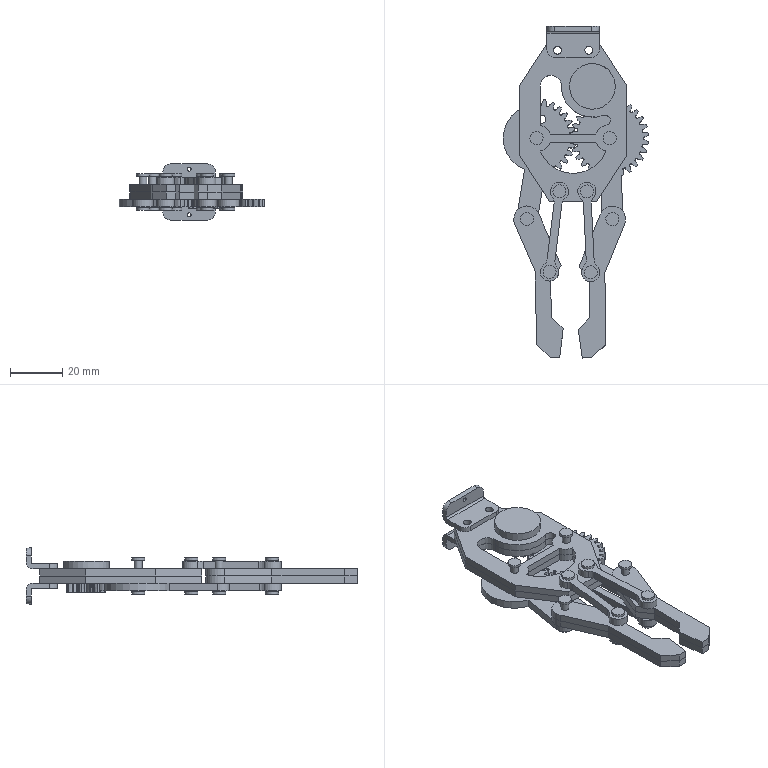Assembly | NX | mm | 23 component files | 23 solids | 679 faces | box 55.7 x 126.98 x 21.44 mm | volume 22522 mm3 | cylinder 325 | plane 246 | other 108 | commonest cylinder face diameters 0.5 x101 3 x46 30 x39 25.5 x38 6 x20 5 x16 15 x13 10.5 x13
Bill of materials:
unnamed part 1 | 1 |  | Short cylindrical part with a thin, flat, circular head on top of a slightly smaller shank that has lengthwise ribs or flutes around its outside.
unnamed part 2 | 2 |  | L-shaped bracket. A flat flange with two holes bends 90 degrees into a shorter leg with one smaller hole.
unnamed part 3 | 8 |  | Spool- or pin-like part: a straight cylindrical shaft with a thin, larger-diameter flat flange at each end.
unnamed part 4 | 1 |  | Flat spur-gear-like disc with teeth all the way around, a central round hole, and a straight arm extending outward that ends in a rounded tip with a small hole.
unnamed part 5 | 4 |  | Flat link or connecting bar: a narrow straight strip with a round boss at each end, each with a through-hole. Smooth fillets join the bosses to the strip.
unnamed part 6 | 1 |  | Flat plate shaped like a gear sector with an integral arm. Teeth cover only part of the circular edge. There are three holes in a row on the round body and one hole at the rounded end of the arm.
unnamed part 7 | 4 |  | Flat lever-like plate made of two straight segments meeting at an angle. One end is rounded and has a hole. A second hole sits near the angled joint, and the other end narrows to an angled, chamfered tip.
unnamed part 8 | 2 |  | Thin, flat, elongated octagonal plate with several cutouts: a large circular opening, a curved slot that joins it, a D-shaped opening, a narrow bridge between two holes, and eight small round holes.
Mates:
1. fix | BASE-PLATE 2 component
2. bond | BASE-PLATE 2 component | assembly component
3. bond | assembly component
4. linear | assembly datumaxis | assembly cartesiancoordinatesystem | assembly cartesiancoordinatesystem
5. bond | BASE-PLATE 2 component | assembly component
6. touch align | BASE-PLATE 1 face | BASE-PLATE 2 face
7. touch align | BASE-PLATE 1 face | BASE-PLATE 2 face
8. touch align | BASE-PLATE 1 face | BASE-PLATE 2 face
9. touch align | BASE-MOUNTING-BRACKET 2 face | BASE-PLATE 1 face
10. touch align | BASE-MOUNTING-BRACKET 2 face | BASE-PLATE 1 face
11. touch align | BASE-MOUNTING-BRACKET 2 face | BASE-PLATE 1 face
12. touch align | BASE-MOUNTING-BRACKET 1 face | BASE-PLATE 2 face
13. touch align | BASE-MOUNTING-BRACKET 1 face | BASE-PLATE 2 face
14. touch align | BASE-MOUNTING-BRACKET 1 face | BASE-PLATE 2 face
15. touch align | LINK 4 face | BASE-PLATE 1 face
16. touch align | LINK 4 face | BASE-PLATE 1 face
17. touch align | LINK 3 face | BASE-PLATE 1 face
18. touch align | LINK 3 face | BASE-PLATE 1 face
19. touch align | LINK 2 face | BASE-PLATE 2 face
20. touch align | LINK 1 face | BASE-PLATE 2 face
21. touch align | BASE-PLATE 2 face | LINK 2 face
22. touch align | GRIPPER 3 face | GRIPPER 4 face
23. touch align | GRIPPER 3 face | GRIPPER 4 face
24. touch align | GRIPPER 3 face | GRIPPER 4 face
25. touch align | GRIPPER 3 face | LINK 4 face
26. touch align | LINK 1 face | GRIPPER 4 face
27. touch align | GRIPPER 1 face | GRIPPER 2 face
28. touch align | LINK 3 face | GRIPPER 2 face
29. touch align | LINK 2 face | GRIPPER 1 face
30. touch align | PIN 2 face | LINK 3 face
31. distance | LINK 3 face | PIN 2 face
32. touch align | PIN 3 face | LINK 3 face
33. distance | PIN 3 face | LINK 2 face
34. touch align | PIN 1 face | LINK 4 face
35. distance | PIN 1 face | LINK 1 face
36. touch align | PIN 6 face | LINK 1 face
37. distance | PIN 6 face | LINK 1 face
38. touch align | PIN 7 face | GRIPPER 1 face
39. touch align | PIN 8 face | BASE-PLATE 2 face
40. touch align | PIN 4 face | GRIPPER 4 face
41. touch align | PIN 5 face | BASE-PLATE 2 face
42. touch align | BASE-GEAR-YENI 1 face | BASE-PLATE 1 face
43. touch align | BASE-GEAR-YENI 1 edge | BASE-PLATE 1 edge
44. touch align | GEAR-LINK-2_yen 1 face | BASE-PLATE 2 face
45. touch align | BASE-PLATE 2 face | GEAR-LINK-1_yen 1 face
46. touch align | GEAR-LINK-1_yen 1 face | PIN 8 face
47. touch align | GEAR-LINK-1_yen 1 face | PIN 7 face
48. touch align | PIN 6 face | BASE-PLATE 2 face
49. touch align | GEAR-LINK-2_yen 1 face | PIN 4 face
50. touch align | GEAR-LINK-2_yen 1 face | PIN 5 face